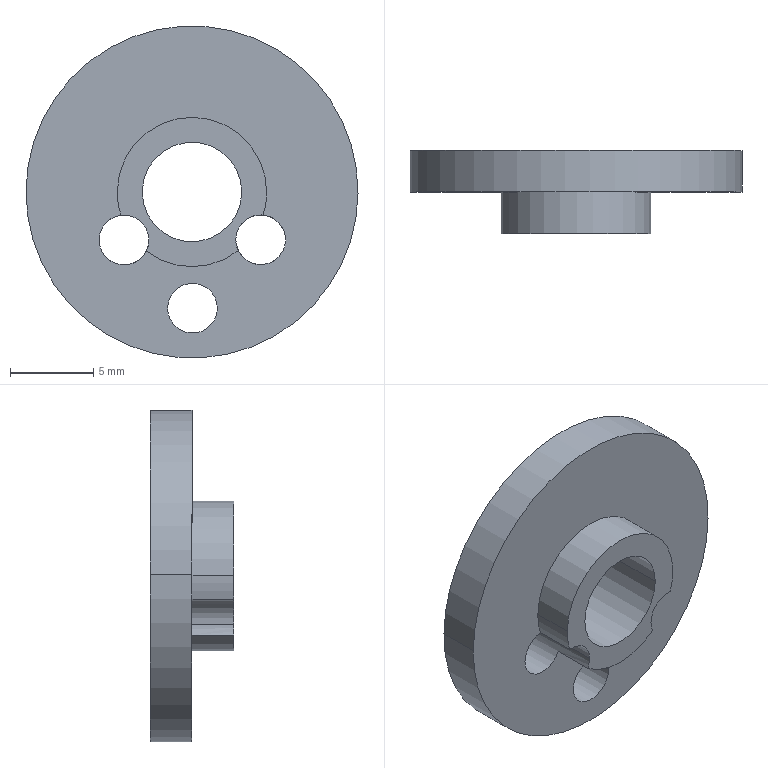Component | SolidWorks | Part6-1 | 1 solid | 17 faces | box 20 x 5 x 20 mm | volume 741 mm3 | cylinder 14 | plane 3 | commonest cylinder face diameters 3 x6 9 x4 20 x2 6 x2 | material 45
build123d program:
from build123d import *

# Parameters (mm, degrees)
SKETCH3_R                = 4.5
SKETCH3_R_2              = 3
BOSS_EXTRUDE1_DEPTH      = 3
BOSS_EXTRUDE2_DEPTH      = 2
BOSS_EXTRUDE2_DEPTH_BACK = 0.5
SKETCH4_R                = 10
SKETCH4_R_2              = 3
SKETCH5_R                = 1.5
CUT_EXTRUDE1_DEPTH       = 16


with BuildPart() as part:
    # Sketch3 → Boss-Extrude1 (new body)
    with BuildSketch(Plane.XY):
        Circle(SKETCH3_R)
        Circle(SKETCH3_R_2, mode=Mode.SUBTRACT)
    extrude(amount=BOSS_EXTRUDE1_DEPTH)

    # Sketch4 → Boss-Extrude2 (add, two sides: drawn at the far end of the back side and taken through both)
    with BuildSketch(Plane.XY.offset(3).offset(-BOSS_EXTRUDE2_DEPTH_BACK)):
        Circle(SKETCH4_R)
        Circle(SKETCH4_R_2, mode=Mode.SUBTRACT)
    extrude(amount=BOSS_EXTRUDE2_DEPTH + BOSS_EXTRUDE2_DEPTH_BACK)

    # Sketch5 → Cut-Extrude1 (cut, through all)
    with BuildSketch(Plane.XY.offset(5)):
        with Locations((4.165, 2.835)):
            Circle(SKETCH5_R)
        with Locations((0.09793, 7)):
            Circle(SKETCH5_R)
        with Locations((0, -1.232)):
            Circle(SKETCH5_R)
        with Locations((-4.067, 2.933)):
            Circle(SKETCH5_R)
    extrude(amount=-CUT_EXTRUDE1_DEPTH, mode=Mode.SUBTRACT)


solid = part.part

# Placed as in the assembly
solid = solid.moved(Location((0, 12.25, 0), (-90, 0, 0.5611)))
STEP:
#1=COLOUR_RGB('',0.7922,0.8196,0.9333);
#2=FILL_AREA_STYLE_COLOUR('',#1);
#3=FILL_AREA_STYLE('',(#2));
#4=SURFACE_STYLE_FILL_AREA(#3);
#5=SURFACE_SIDE_STYLE('',(#4));
#6=SURFACE_STYLE_USAGE(.BOTH.,#5);
#7=PRESENTATION_STYLE_ASSIGNMENT((#6));
#8=CARTESIAN_POINT('',(-0.2203,0.5807,-0.1133));
#9=VERTEX_POINT('',#8);
#10=CARTESIAN_POINT('',(-0.1683,0.5807,-0.05527));
#11=VERTEX_POINT('',#10);
#12=CARTESIAN_POINT('',(-0.1612,0.5807,-0.1139));
#13=DIRECTION('',(-0.,1.,0.));
#14=DIRECTION('',(1.,0.,-0.009793));
#15=AXIS2_PLACEMENT_3D('',#12,#13,#14);
#16=CIRCLE('',#15,0.05906);
#17=EDGE_CURVE('',#9,#11,#16,.T.);
#18=ORIENTED_EDGE('',*,*,#17,.F.);
#19=CARTESIAN_POINT('',(-0.2203,0.6791,-0.1133));
#20=VERTEX_POINT('',#19);
#21=CARTESIAN_POINT('',(-0.2203,0.4823,-0.1133));
#22=DIRECTION('',(-0.,1.,0.));
#23=VECTOR('',#22,39.37);
#24=LINE('',#21,#23);
#25=EDGE_CURVE('',#9,#20,#24,.T.);
#26=ORIENTED_EDGE('',*,*,#25,.T.);
#27=CARTESIAN_POINT('',(-0.1022,0.6791,-0.1145));
#28=VERTEX_POINT('',#27);
#29=CARTESIAN_POINT('',(-0.1612,0.6791,-0.1139));
#30=DIRECTION('',(-0.,1.,0.));
#31=DIRECTION('',(1.,0.,-0.009793));
#32=AXIS2_PLACEMENT_3D('',#29,#30,#31);
#33=CIRCLE('',#32,0.05906);
#34=EDGE_CURVE('',#20,#28,#33,.T.);
#35=ORIENTED_EDGE('',*,*,#34,.T.);
#36=CARTESIAN_POINT('',(-0.1022,0.4823,-0.1145));
#37=VERTEX_POINT('',#36);
#38=CARTESIAN_POINT('',(-0.1022,0.4823,-0.1145));
#39=DIRECTION('',(-0.,1.,0.));
#40=VECTOR('',#39,39.37);
#41=LINE('',#38,#40);
#42=EDGE_CURVE('',#37,#28,#41,.T.);
#43=ORIENTED_EDGE('',*,*,#42,.F.);
#44=CARTESIAN_POINT('',(-0.1683,0.4823,-0.05527));
#45=VERTEX_POINT('',#44);
#46=CARTESIAN_POINT('',(-0.1612,0.4823,-0.1139));
#47=DIRECTION('',(-0.,1.,0.));
#48=DIRECTION('',(1.,0.,-0.009793));
#49=AXIS2_PLACEMENT_3D('',#46,#47,#48);
#50=CIRCLE('',#49,0.05906);
#51=EDGE_CURVE('',#45,#37,#50,.T.);
#52=ORIENTED_EDGE('',*,*,#51,.F.);
#53=CARTESIAN_POINT('',(-0.1683,0.5807,-0.05527));
#54=DIRECTION('',(0.,-1.,-0.));
#55=VECTOR('',#54,39.37);
#56=LINE('',#53,#55);
#57=EDGE_CURVE('',#11,#45,#56,.T.);
#58=ORIENTED_EDGE('',*,*,#57,.F.);
#59=EDGE_LOOP('',(#18,#26,#35,#43,#52,#58));
#60=FACE_OUTER_BOUND('',#59,.T.);
#61=CARTESIAN_POINT('',(-0.1612,0.4823,-0.1139));
#62=DIRECTION('',(-0.,1.,0.));
#63=DIRECTION('',(1.,0.,-0.009793));
#64=AXIS2_PLACEMENT_3D('',#61,#62,#63);
#65=CYLINDRICAL_SURFACE('',#64,0.05906);
#66=ADVANCED_FACE('',(#60),#65,.F.);
#67=CARTESIAN_POINT('',(0.1038,0.4823,-0.1126));
#68=VERTEX_POINT('',#67);
#69=CARTESIAN_POINT('',(0.1686,0.4823,-0.05444));
#70=VERTEX_POINT('',#69);
#71=CARTESIAN_POINT('',(0.1629,0.4823,-0.1132));
#72=DIRECTION('',(-0.,1.,0.));
#73=DIRECTION('',(1.,0.,-0.009793));
#74=AXIS2_PLACEMENT_3D('',#71,#72,#73);
#75=CIRCLE('',#74,0.05906);
#76=EDGE_CURVE('',#68,#70,#75,.T.);
#77=ORIENTED_EDGE('',*,*,#76,.F.);
#78=CARTESIAN_POINT('',(0.1038,0.6791,-0.1126));
#79=VERTEX_POINT('',#78);
#80=CARTESIAN_POINT('',(0.1038,0.4823,-0.1126));
#81=DIRECTION('',(-0.,1.,0.));
#82=VECTOR('',#81,39.37);
#83=LINE('',#80,#82);
#84=EDGE_CURVE('',#68,#79,#83,.T.);
#85=ORIENTED_EDGE('',*,*,#84,.T.);
#86=CARTESIAN_POINT('',(0.2219,0.6791,-0.1138));
#87=VERTEX_POINT('',#86);
#88=CARTESIAN_POINT('',(0.1629,0.6791,-0.1132));
#89=DIRECTION('',(-0.,1.,0.));
#90=DIRECTION('',(1.,0.,-0.009793));
#91=AXIS2_PLACEMENT_3D('',#88,#89,#90);
#92=CIRCLE('',#91,0.05906);
#93=EDGE_CURVE('',#79,#87,#92,.T.);
#94=ORIENTED_EDGE('',*,*,#93,.T.);
#95=CARTESIAN_POINT('',(0.2219,0.5807,-0.1138));
#96=VERTEX_POINT('',#95);
#97=CARTESIAN_POINT('',(0.2219,0.4823,-0.1138));
#98=DIRECTION('',(-0.,1.,0.));
#99=VECTOR('',#98,39.37);
#100=LINE('',#97,#99);
#101=EDGE_CURVE('',#96,#87,#100,.T.);
#102=ORIENTED_EDGE('',*,*,#101,.F.);
#103=CARTESIAN_POINT('',(0.1686,0.5807,-0.05444));
#104=VERTEX_POINT('',#103);
#105=CARTESIAN_POINT('',(0.1629,0.5807,-0.1132));
#106=DIRECTION('',(-0.,1.,0.));
#107=DIRECTION('',(1.,0.,-0.009793));
#108=AXIS2_PLACEMENT_3D('',#105,#106,#107);
#109=CIRCLE('',#108,0.05906);
#110=EDGE_CURVE('',#104,#96,#109,.T.);
#111=ORIENTED_EDGE('',*,*,#110,.F.);
#112=CARTESIAN_POINT('',(0.1686,0.5807,-0.05444));
#113=DIRECTION('',(-0.,1.,0.));
#114=VECTOR('',#113,39.37);
#115=LINE('',#112,#114);
#116=EDGE_CURVE('',#70,#104,#115,.T.);
#117=ORIENTED_EDGE('',*,*,#116,.F.);
#118=EDGE_LOOP('',(#77,#85,#94,#102,#111,#117));
#119=FACE_OUTER_BOUND('',#118,.T.);
#120=CARTESIAN_POINT('',(0.1629,0.4823,-0.1132));
#121=DIRECTION('',(-0.,1.,0.));
#122=DIRECTION('',(1.,0.,-0.009793));
#123=AXIS2_PLACEMENT_3D('',#120,#121,#122);
#124=CYLINDRICAL_SURFACE('',#123,0.05906);
#125=ADVANCED_FACE('',(#119),#124,.F.);
#126=CARTESIAN_POINT('',(-0.0579,0.5807,-0.275));
#127=VERTEX_POINT('',#126);
#128=CARTESIAN_POINT('',(0.06021,0.5807,-0.2762));
#129=VERTEX_POINT('',#128);
#130=CARTESIAN_POINT('',(0.001157,0.5807,-0.2756));
#131=DIRECTION('',(-0.,1.,0.));
#132=DIRECTION('',(1.,0.,-0.009793));
#133=AXIS2_PLACEMENT_3D('',#130,#131,#132);
#134=CIRCLE('',#133,0.05906);
#135=EDGE_CURVE('',#127,#129,#134,.T.);
#136=ORIENTED_EDGE('',*,*,#135,.F.);
#137=CARTESIAN_POINT('',(-0.0579,0.6791,-0.275));
#138=VERTEX_POINT('',#137);
#139=CARTESIAN_POINT('',(-0.0579,0.4823,-0.275));
#140=DIRECTION('',(-0.,1.,0.));
#141=VECTOR('',#140,39.37);
#142=LINE('',#139,#141);
#143=EDGE_CURVE('',#127,#138,#142,.T.);
#144=ORIENTED_EDGE('',*,*,#143,.T.);
#145=CARTESIAN_POINT('',(0.06021,0.6791,-0.2762));
#146=VERTEX_POINT('',#145);
#147=CARTESIAN_POINT('',(0.001157,0.6791,-0.2756));
#148=DIRECTION('',(-0.,1.,0.));
#149=DIRECTION('',(1.,0.,-0.009793));
#150=AXIS2_PLACEMENT_3D('',#147,#148,#149);
#151=CIRCLE('',#150,0.05906);
#152=EDGE_CURVE('',#138,#146,#151,.T.);
#153=ORIENTED_EDGE('',*,*,#152,.T.);
#154=CARTESIAN_POINT('',(0.06021,0.4823,-0.2762));
#155=DIRECTION('',(-0.,1.,0.));
#156=VECTOR('',#155,39.37);
#157=LINE('',#154,#156);
#158=EDGE_CURVE('',#129,#146,#157,.T.);
#159=ORIENTED_EDGE('',*,*,#158,.F.);
#160=EDGE_LOOP('',(#136,#144,#153,#159));
#161=FACE_OUTER_BOUND('',#160,.T.);
#162=CARTESIAN_POINT('',(0.001157,0.4823,-0.2756));
#163=DIRECTION('',(-0.,1.,0.));
#164=DIRECTION('',(1.,0.,-0.009793));
#165=AXIS2_PLACEMENT_3D('',#162,#163,#164);
#166=CYLINDRICAL_SURFACE('',#165,0.05906);
#167=ADVANCED_FACE('',(#161),#166,.F.);
#168=CARTESIAN_POINT('',(0.3937,0.5807,-0.003856));
#169=VERTEX_POINT('',#168);
#170=CARTESIAN_POINT('',(-0.3937,0.5807,0.003856));
#171=VERTEX_POINT('',#170);
#172=CARTESIAN_POINT('',(-0.,0.5807,-0.));
#173=DIRECTION('',(-0.,1.,0.));
#174=DIRECTION('',(1.,0.,-0.009793));
#175=AXIS2_PLACEMENT_3D('',#172,#173,#174);
#176=CIRCLE('',#175,0.3937);
#177=EDGE_CURVE('',#169,#171,#176,.T.);
#178=ORIENTED_EDGE('',*,*,#177,.T.);
#179=CARTESIAN_POINT('',(-0.3937,0.6791,0.003856));
#180=VERTEX_POINT('',#179);
#181=CARTESIAN_POINT('',(-0.3937,0.5807,0.003856));
#182=DIRECTION('',(-0.,1.,0.));
#183=VECTOR('',#182,39.37);
#184=LINE('',#181,#183);
#185=EDGE_CURVE('',#171,#180,#184,.T.);
#186=ORIENTED_EDGE('',*,*,#185,.T.);
#187=CARTESIAN_POINT('',(0.3937,0.6791,-0.003856));
#188=VERTEX_POINT('',#187);
#189=CARTESIAN_POINT('',(-0.,0.6791,-0.));
#190=DIRECTION('',(-0.,1.,0.));
#191=DIRECTION('',(1.,0.,-0.009793));
#192=AXIS2_PLACEMENT_3D('',#189,#190,#191);
#193=CIRCLE('',#192,0.3937);
#194=EDGE_CURVE('',#188,#180,#193,.T.);
#195=ORIENTED_EDGE('',*,*,#194,.F.);
#196=CARTESIAN_POINT('',(0.3937,0.5807,-0.003856));
#197=DIRECTION('',(-0.,1.,0.));
#198=VECTOR('',#197,39.37);
#199=LINE('',#196,#198);
#200=EDGE_CURVE('',#169,#188,#199,.T.);
#201=ORIENTED_EDGE('',*,*,#200,.F.);
#202=EDGE_LOOP('',(#178,#186,#195,#201));
#203=FACE_OUTER_BOUND('',#202,.T.);
#204=CARTESIAN_POINT('',(-0.,0.5807,-0.));
#205=DIRECTION('',(-0.,1.,0.));
#206=DIRECTION('',(1.,0.,-0.009793));
#207=AXIS2_PLACEMENT_3D('',#204,#205,#206);
#208=CYLINDRICAL_SURFACE('',#207,0.3937);
#209=ADVANCED_FACE('',(#203),#208,.T.);
#210=CARTESIAN_POINT('',(-0.1181,0.6791,0.001157));
#211=VERTEX_POINT('',#210);
#212=CARTESIAN_POINT('',(0.1181,0.6791,-0.001157));
#213=VERTEX_POINT('',#212);
#214=CARTESIAN_POINT('',(-0.,0.6791,-0.));
#215=DIRECTION('',(-0.,1.,0.));
#216=DIRECTION('',(1.,0.,-0.009793));
#217=AXIS2_PLACEMENT_3D('',#214,#215,#216);
#218=CIRCLE('',#217,0.1181);
#219=EDGE_CURVE('',#211,#213,#218,.T.);
#220=ORIENTED_EDGE('',*,*,#219,.T.);
#221=CARTESIAN_POINT('',(0.1181,0.4823,-0.001157));
#222=VERTEX_POINT('',#221);
#223=CARTESIAN_POINT('',(0.1181,0.6004,-0.001157));
#224=DIRECTION('',(0.,-1.,-0.));
#225=VECTOR('',#224,39.37);
#226=LINE('',#223,#225);
#227=EDGE_CURVE('',#213,#222,#226,.T.);
#228=ORIENTED_EDGE('',*,*,#227,.T.);
#229=CARTESIAN_POINT('',(-0.1181,0.4823,0.001157));
#230=VERTEX_POINT('',#229);
#231=CARTESIAN_POINT('',(-0.,0.4823,-0.));
#232=DIRECTION('',(-0.,1.,0.));
#233=DIRECTION('',(1.,0.,-0.009793));
#234=AXIS2_PLACEMENT_3D('',#231,#232,#233);
#235=CIRCLE('',#234,0.1181);
#236=EDGE_CURVE('',#230,#222,#235,.T.);
#237=ORIENTED_EDGE('',*,*,#236,.F.);
#238=CARTESIAN_POINT('',(-0.1181,0.6004,0.001157));
#239=DIRECTION('',(0.,-1.,-0.));
#240=VECTOR('',#239,39.37);
#241=LINE('',#238,#240);
#242=EDGE_CURVE('',#211,#230,#241,.T.);
#243=ORIENTED_EDGE('',*,*,#242,.F.);
#244=EDGE_LOOP('',(#220,#228,#237,#243));
#245=FACE_OUTER_BOUND('',#244,.T.);
#246=CARTESIAN_POINT('',(-0.,0.6004,-0.));
#247=DIRECTION('',(0.,-1.,-0.));
#248=DIRECTION('',(-1.,0.,0.009793));
#249=AXIS2_PLACEMENT_3D('',#246,#247,#248);
#250=CYLINDRICAL_SURFACE('',#249,0.1181);
#251=ADVANCED_FACE('',(#245),#250,.F.);
#252=CARTESIAN_POINT('',(0.1772,0.5807,-0.001735));
#253=VERTEX_POINT('',#252);
#254=CARTESIAN_POINT('',(-0.,0.5807,-0.));
#255=DIRECTION('',(-0.,1.,0.));
#256=DIRECTION('',(1.,0.,-0.009793));
#257=AXIS2_PLACEMENT_3D('',#254,#255,#256);
#258=CIRCLE('',#257,0.1772);
#259=EDGE_CURVE('',#253,#104,#258,.T.);
#260=ORIENTED_EDGE('',*,*,#259,.F.);
#261=CARTESIAN_POINT('',(0.1772,0.4823,-0.001735));
#262=VERTEX_POINT('',#261);
#263=CARTESIAN_POINT('',(0.1772,0.6004,-0.001735));
#264=DIRECTION('',(0.,-1.,-0.));
#265=VECTOR('',#264,39.37);
#266=LINE('',#263,#265);
#267=EDGE_CURVE('',#253,#262,#266,.T.);
#268=ORIENTED_EDGE('',*,*,#267,.T.);
#269=CARTESIAN_POINT('',(-0.,0.4823,-0.));
#270=DIRECTION('',(-0.,1.,0.));
#271=DIRECTION('',(1.,0.,-0.009793));
#272=AXIS2_PLACEMENT_3D('',#269,#270,#271);
#273=CIRCLE('',#272,0.1772);
#274=EDGE_CURVE('',#262,#70,#273,.T.);
#275=ORIENTED_EDGE('',*,*,#274,.T.);
#276=ORIENTED_EDGE('',*,*,#116,.T.);
#277=EDGE_LOOP('',(#260,#268,#275,#276));
#278=FACE_OUTER_BOUND('',#277,.T.);
#279=CARTESIAN_POINT('',(-0.,0.6004,-0.));
#280=DIRECTION('',(0.,-1.,-0.));
#281=DIRECTION('',(-1.,0.,0.009793));
#282=AXIS2_PLACEMENT_3D('',#279,#280,#281);
#283=CYLINDRICAL_SURFACE('',#282,0.1772);
#284=ADVANCED_FACE('',(#278),#283,.T.);
#285=ORIENTED_EDGE('',*,*,#267,.F.);
#286=CARTESIAN_POINT('',(-0.1772,0.5807,0.001735));
#287=VERTEX_POINT('',#286);
#288=CARTESIAN_POINT('',(-0.,0.5807,-0.));
#289=DIRECTION('',(-0.,1.,0.));
#290=DIRECTION('',(1.,0.,-0.009793));
#291=AXIS2_PLACEMENT_3D('',#288,#289,#290);
#292=CIRCLE('',#291,0.1772);
#293=EDGE_CURVE('',#287,#253,#292,.T.);
#294=ORIENTED_EDGE('',*,*,#293,.F.);
#295=CARTESIAN_POINT('',(-0.1772,0.4823,0.001735));
#296=VERTEX_POINT('',#295);
#297=CARTESIAN_POINT('',(-0.1772,0.6004,0.001735));
#298=DIRECTION('',(0.,-1.,-0.));
#299=VECTOR('',#298,39.37);
#300=LINE('',#297,#299);
#301=EDGE_CURVE('',#287,#296,#300,.T.);
#302=ORIENTED_EDGE('',*,*,#301,.T.);
#303=CARTESIAN_POINT('',(-0.,0.4823,-0.));
#304=DIRECTION('',(-0.,1.,0.));
#305=DIRECTION('',(1.,0.,-0.009793));
#306=AXIS2_PLACEMENT_3D('',#303,#304,#305);
#307=CIRCLE('',#306,0.1772);
#308=EDGE_CURVE('',#296,#262,#307,.T.);
#309=ORIENTED_EDGE('',*,*,#308,.T.);
#310=EDGE_LOOP('',(#285,#294,#302,#309));
#311=FACE_OUTER_BOUND('',#310,.T.);
#312=CARTESIAN_POINT('',(-0.,0.6004,-0.));
#313=DIRECTION('',(0.,-1.,-0.));
#314=DIRECTION('',(-1.,0.,0.009793));
#315=AXIS2_PLACEMENT_3D('',#312,#313,#314);
#316=CYLINDRICAL_SURFACE('',#315,0.1772);
#317=ADVANCED_FACE('',(#311),#316,.T.);
#318=CARTESIAN_POINT('',(0.1098,0.4823,-0.1391));
#319=VERTEX_POINT('',#318);
#320=CARTESIAN_POINT('',(-0.1084,0.4823,-0.1402));
#321=VERTEX_POINT('',#320);
#322=CARTESIAN_POINT('',(-0.,0.4823,-0.));
#323=DIRECTION('',(-0.,1.,0.));
#324=DIRECTION('',(1.,0.,-0.009793));
#325=AXIS2_PLACEMENT_3D('',#322,#323,#324);
#326=CIRCLE('',#325,0.1772);
#327=EDGE_CURVE('',#319,#321,#326,.T.);
#328=ORIENTED_EDGE('',*,*,#327,.T.);
#329=CARTESIAN_POINT('',(-0.1084,0.5807,-0.1402));
#330=VERTEX_POINT('',#329);
#331=CARTESIAN_POINT('',(-0.1084,0.5807,-0.1402));
#332=DIRECTION('',(-0.,1.,0.));
#333=VECTOR('',#332,39.37);
#334=LINE('',#331,#333);
#335=EDGE_CURVE('',#321,#330,#334,.T.);
#336=ORIENTED_EDGE('',*,*,#335,.T.);
#337=CARTESIAN_POINT('',(0.1098,0.5807,-0.1391));
#338=VERTEX_POINT('',#337);
#339=CARTESIAN_POINT('',(-0.,0.5807,-0.));
#340=DIRECTION('',(-0.,1.,0.));
#341=DIRECTION('',(1.,0.,-0.009793));
#342=AXIS2_PLACEMENT_3D('',#339,#340,#341);
#343=CIRCLE('',#342,0.1772);
#344=EDGE_CURVE('',#338,#330,#343,.T.);
#345=ORIENTED_EDGE('',*,*,#344,.F.);
#346=CARTESIAN_POINT('',(0.1098,0.5807,-0.1391));
#347=DIRECTION('',(0.,-1.,-0.));
#348=VECTOR('',#347,39.37);
#349=LINE('',#346,#348);
#350=EDGE_CURVE('',#338,#319,#349,.T.);
#351=ORIENTED_EDGE('',*,*,#350,.T.);
#352=EDGE_LOOP('',(#328,#336,#345,#351));
#353=FACE_OUTER_BOUND('',#352,.T.);
#354=CARTESIAN_POINT('',(-0.,0.6004,-0.));
#355=DIRECTION('',(0.,-1.,-0.));
#356=DIRECTION('',(-1.,0.,0.009793));
#357=AXIS2_PLACEMENT_3D('',#354,#355,#356);
#358=CYLINDRICAL_SURFACE('',#357,0.1772);
#359=ADVANCED_FACE('',(#353),#358,.T.);
#360=ORIENTED_EDGE('',*,*,#301,.F.);
#361=CARTESIAN_POINT('',(-0.,0.5807,-0.));
#362=DIRECTION('',(-0.,1.,0.));
#363=DIRECTION('',(1.,0.,-0.009793));
#364=AXIS2_PLACEMENT_3D('',#361,#362,#363);
#365=CIRCLE('',#364,0.1772);
#366=EDGE_CURVE('',#11,#287,#365,.T.);
#367=ORIENTED_EDGE('',*,*,#366,.F.);
#368=ORIENTED_EDGE('',*,*,#57,.T.);
#369=CARTESIAN_POINT('',(-0.,0.4823,-0.));
#370=DIRECTION('',(-0.,1.,0.));
#371=DIRECTION('',(1.,0.,-0.009793));
#372=AXIS2_PLACEMENT_3D('',#369,#370,#371);
#373=CIRCLE('',#372,0.1772);
#374=EDGE_CURVE('',#45,#296,#373,.T.);
#375=ORIENTED_EDGE('',*,*,#374,.T.);
#376=EDGE_LOOP('',(#360,#367,#368,#375));
#377=FACE_OUTER_BOUND('',#376,.T.);
#378=CARTESIAN_POINT('',(-0.,0.6004,-0.));
#379=DIRECTION('',(0.,-1.,-0.));
#380=DIRECTION('',(-1.,0.,0.009793));
#381=AXIS2_PLACEMENT_3D('',#378,#379,#380);
#382=CYLINDRICAL_SURFACE('',#381,0.1772);
#383=ADVANCED_FACE('',(#377),#382,.T.);
#384=ORIENTED_EDGE('',*,*,#374,.F.);
#385=ORIENTED_EDGE('',*,*,#51,.T.);
#386=CARTESIAN_POINT('',(-0.1612,0.4823,-0.1139));
#387=DIRECTION('',(-0.,1.,0.));
#388=DIRECTION('',(1.,0.,-0.009793));
#389=AXIS2_PLACEMENT_3D('',#386,#387,#388);
#390=CIRCLE('',#389,0.05906);
#391=EDGE_CURVE('',#37,#321,#390,.T.);
#392=ORIENTED_EDGE('',*,*,#391,.T.);
#393=ORIENTED_EDGE('',*,*,#327,.F.);
#394=CARTESIAN_POINT('',(0.1629,0.4823,-0.1132));
#395=DIRECTION('',(-0.,1.,0.));
#396=DIRECTION('',(1.,0.,-0.009793));
#397=AXIS2_PLACEMENT_3D('',#394,#395,#396);
#398=CIRCLE('',#397,0.05906);
#399=EDGE_CURVE('',#319,#68,#398,.T.);
#400=ORIENTED_EDGE('',*,*,#399,.T.);
#401=ORIENTED_EDGE('',*,*,#76,.T.);
#402=ORIENTED_EDGE('',*,*,#274,.F.);
#403=ORIENTED_EDGE('',*,*,#308,.F.);
#404=EDGE_LOOP('',(#384,#385,#392,#393,#400,#401,#402,#403));
#405=FACE_OUTER_BOUND('',#404,.T.);
#406=ORIENTED_EDGE('',*,*,#236,.T.);
#407=CARTESIAN_POINT('',(-0.,0.4823,-0.));
#408=DIRECTION('',(-0.,1.,0.));
#409=DIRECTION('',(1.,0.,-0.009793));
#410=AXIS2_PLACEMENT_3D('',#407,#408,#409);
#411=CIRCLE('',#410,0.1181);
#412=EDGE_CURVE('',#222,#230,#411,.T.);
#413=ORIENTED_EDGE('',*,*,#412,.T.);
#414=EDGE_LOOP('',(#406,#413));
#415=FACE_BOUND('',#414,.T.);
#416=CARTESIAN_POINT('',(-0.,0.4823,-0.));
#417=DIRECTION('',(-0.,1.,0.));
#418=DIRECTION('',(1.,0.,-0.009793));
#419=AXIS2_PLACEMENT_3D('',#416,#417,#418);
#420=PLANE('',#419);
#421=ADVANCED_FACE('',(#405,#415),#420,.F.);
#422=ORIENTED_EDGE('',*,*,#227,.F.);
#423=CARTESIAN_POINT('',(-0.,0.6791,-0.));
#424=DIRECTION('',(-0.,1.,0.));
#425=DIRECTION('',(1.,0.,-0.009793));
#426=AXIS2_PLACEMENT_3D('',#423,#424,#425);
#427=CIRCLE('',#426,0.1181);
#428=EDGE_CURVE('',#213,#211,#427,.T.);
#429=ORIENTED_EDGE('',*,*,#428,.T.);
#430=ORIENTED_EDGE('',*,*,#242,.T.);
#431=ORIENTED_EDGE('',*,*,#412,.F.);
#432=EDGE_LOOP('',(#422,#429,#430,#431));
#433=FACE_OUTER_BOUND('',#432,.T.);
#434=CARTESIAN_POINT('',(-0.,0.6004,-0.));
#435=DIRECTION('',(0.,-1.,-0.));
#436=DIRECTION('',(-1.,0.,0.009793));
#437=AXIS2_PLACEMENT_3D('',#434,#435,#436);
#438=CYLINDRICAL_SURFACE('',#437,0.1181);
#439=ADVANCED_FACE('',(#433),#438,.F.);
#440=CARTESIAN_POINT('',(0.001157,0.5807,-0.2756));
#441=DIRECTION('',(-0.,1.,0.));
#442=DIRECTION('',(1.,0.,-0.009793));
#443=AXIS2_PLACEMENT_3D('',#440,#441,#442);
#444=CIRCLE('',#443,0.05906);
#445=EDGE_CURVE('',#129,#127,#444,.T.);
#446=ORIENTED_EDGE('',*,*,#445,.T.);
#447=ORIENTED_EDGE('',*,*,#135,.T.);
#448=EDGE_LOOP('',(#446,#447));
#449=FACE_BOUND('',#448,.T.);
#450=ORIENTED_EDGE('',*,*,#177,.F.);
#451=CARTESIAN_POINT('',(-0.,0.5807,-0.));
#452=DIRECTION('',(-0.,1.,0.));
#453=DIRECTION('',(1.,0.,-0.009793));
#454=AXIS2_PLACEMENT_3D('',#451,#452,#453);
#455=CIRCLE('',#454,0.3937);
#456=EDGE_CURVE('',#171,#169,#455,.T.);
#457=ORIENTED_EDGE('',*,*,#456,.F.);
#458=EDGE_LOOP('',(#450,#457));
#459=FACE_OUTER_BOUND('',#458,.T.);
#460=ORIENTED_EDGE('',*,*,#344,.T.);
#461=CARTESIAN_POINT('',(-0.1612,0.5807,-0.1139));
#462=DIRECTION('',(-0.,1.,0.));
#463=DIRECTION('',(1.,0.,-0.009793));
#464=AXIS2_PLACEMENT_3D('',#461,#462,#463);
#465=CIRCLE('',#464,0.05906);
#466=EDGE_CURVE('',#330,#9,#465,.T.);
#467=ORIENTED_EDGE('',*,*,#466,.T.);
#468=ORIENTED_EDGE('',*,*,#17,.T.);
#469=ORIENTED_EDGE('',*,*,#366,.T.);
#470=ORIENTED_EDGE('',*,*,#293,.T.);
#471=ORIENTED_EDGE('',*,*,#259,.T.);
#472=ORIENTED_EDGE('',*,*,#110,.T.);
#473=CARTESIAN_POINT('',(0.1629,0.5807,-0.1132));
#474=DIRECTION('',(-0.,1.,0.));
#475=DIRECTION('',(1.,0.,-0.009793));
#476=AXIS2_PLACEMENT_3D('',#473,#474,#475);
#477=CIRCLE('',#476,0.05906);
#478=EDGE_CURVE('',#96,#338,#477,.T.);
#479=ORIENTED_EDGE('',*,*,#478,.T.);
#480=EDGE_LOOP('',(#460,#467,#468,#469,#470,#471,#472,#479));
#481=FACE_BOUND('',#480,.T.);
#482=CARTESIAN_POINT('',(-0.,0.5807,-0.));
#483=DIRECTION('',(-0.,1.,0.));
#484=DIRECTION('',(1.,0.,-0.009793));
#485=AXIS2_PLACEMENT_3D('',#482,#483,#484);
#486=PLANE('',#485);
#487=ADVANCED_FACE('',(#449,#459,#481),#486,.F.);
#488=ORIENTED_EDGE('',*,*,#185,.F.);
#489=ORIENTED_EDGE('',*,*,#456,.T.);
#490=ORIENTED_EDGE('',*,*,#200,.T.);
#491=CARTESIAN_POINT('',(-0.,0.6791,-0.));
#492=DIRECTION('',(-0.,1.,0.));
#493=DIRECTION('',(1.,0.,-0.009793));
#494=AXIS2_PLACEMENT_3D('',#491,#492,#493);
#495=CIRCLE('',#494,0.3937);
#496=EDGE_CURVE('',#180,#188,#495,.T.);
#497=ORIENTED_EDGE('',*,*,#496,.F.);
#498=EDGE_LOOP('',(#488,#489,#490,#497));
#499=FACE_OUTER_BOUND('',#498,.T.);
#500=CARTESIAN_POINT('',(-0.,0.5807,-0.));
#501=DIRECTION('',(-0.,1.,0.));
#502=DIRECTION('',(1.,0.,-0.009793));
#503=AXIS2_PLACEMENT_3D('',#500,#501,#502);
#504=CYLINDRICAL_SURFACE('',#503,0.3937);
#505=ADVANCED_FACE('',(#499),#504,.T.);
#506=CARTESIAN_POINT('',(-0.1612,0.6791,-0.1139));
#507=DIRECTION('',(-0.,1.,0.));
#508=DIRECTION('',(1.,0.,-0.009793));
#509=AXIS2_PLACEMENT_3D('',#506,#507,#508);
#510=CIRCLE('',#509,0.05906);
#511=EDGE_CURVE('',#28,#20,#510,.T.);
#512=ORIENTED_EDGE('',*,*,#511,.F.);
#513=ORIENTED_EDGE('',*,*,#34,.F.);
#514=EDGE_LOOP('',(#512,#513));
#515=FACE_BOUND('',#514,.T.);
#516=CARTESIAN_POINT('',(0.1629,0.6791,-0.1132));
#517=DIRECTION('',(-0.,1.,0.));
#518=DIRECTION('',(1.,0.,-0.009793));
#519=AXIS2_PLACEMENT_3D('',#516,#517,#518);
#520=CIRCLE('',#519,0.05906);
#521=EDGE_CURVE('',#87,#79,#520,.T.);
#522=ORIENTED_EDGE('',*,*,#521,.F.);
#523=ORIENTED_EDGE('',*,*,#93,.F.);
#524=EDGE_LOOP('',(#522,#523));
#525=FACE_BOUND('',#524,.T.);
#526=CARTESIAN_POINT('',(0.001157,0.6791,-0.2756));
#527=DIRECTION('',(-0.,1.,0.));
#528=DIRECTION('',(1.,0.,-0.009793));
#529=AXIS2_PLACEMENT_3D('',#526,#527,#528);
#530=CIRCLE('',#529,0.05906);
#531=EDGE_CURVE('',#146,#138,#530,.T.);
#532=ORIENTED_EDGE('',*,*,#531,.F.);
#533=ORIENTED_EDGE('',*,*,#152,.F.);
#534=EDGE_LOOP('',(#532,#533));
#535=FACE_BOUND('',#534,.T.);
#536=ORIENTED_EDGE('',*,*,#194,.T.);
#537=ORIENTED_EDGE('',*,*,#496,.T.);
#538=EDGE_LOOP('',(#536,#537));
#539=FACE_OUTER_BOUND('',#538,.T.);
#540=ORIENTED_EDGE('',*,*,#219,.F.);
#541=ORIENTED_EDGE('',*,*,#428,.F.);
#542=EDGE_LOOP('',(#540,#541));
#543=FACE_BOUND('',#542,.T.);
#544=CARTESIAN_POINT('',(-0.,0.6791,-0.));
#545=DIRECTION('',(-0.,1.,0.));
#546=DIRECTION('',(1.,0.,-0.009793));
#547=AXIS2_PLACEMENT_3D('',#544,#545,#546);
#548=PLANE('',#547);
#549=ADVANCED_FACE('',(#515,#525,#535,#539,#543),#548,.T.);
#550=ORIENTED_EDGE('',*,*,#143,.F.);
#551=ORIENTED_EDGE('',*,*,#445,.F.);
#552=ORIENTED_EDGE('',*,*,#158,.T.);
#553=ORIENTED_EDGE('',*,*,#531,.T.);
#554=EDGE_LOOP('',(#550,#551,#552,#553));
#555=FACE_OUTER_BOUND('',#554,.T.);
#556=CARTESIAN_POINT('',(0.001157,0.4823,-0.2756));
#557=DIRECTION('',(-0.,1.,0.));
#558=DIRECTION('',(1.,0.,-0.009793));
#559=AXIS2_PLACEMENT_3D('',#556,#557,#558);
#560=CYLINDRICAL_SURFACE('',#559,0.05906);
#561=ADVANCED_FACE('',(#555),#560,.F.);
#562=ORIENTED_EDGE('',*,*,#84,.F.);
#563=ORIENTED_EDGE('',*,*,#399,.F.);
#564=ORIENTED_EDGE('',*,*,#350,.F.);
#565=ORIENTED_EDGE('',*,*,#478,.F.);
#566=ORIENTED_EDGE('',*,*,#101,.T.);
#567=ORIENTED_EDGE('',*,*,#521,.T.);
#568=EDGE_LOOP('',(#562,#563,#564,#565,#566,#567));
#569=FACE_OUTER_BOUND('',#568,.T.);
#570=CARTESIAN_POINT('',(0.1629,0.4823,-0.1132));
#571=DIRECTION('',(-0.,1.,0.));
#572=DIRECTION('',(1.,0.,-0.009793));
#573=AXIS2_PLACEMENT_3D('',#570,#571,#572);
#574=CYLINDRICAL_SURFACE('',#573,0.05906);
#575=ADVANCED_FACE('',(#569),#574,.F.);
#576=ORIENTED_EDGE('',*,*,#25,.F.);
#577=ORIENTED_EDGE('',*,*,#466,.F.);
#578=ORIENTED_EDGE('',*,*,#335,.F.);
#579=ORIENTED_EDGE('',*,*,#391,.F.);
#580=ORIENTED_EDGE('',*,*,#42,.T.);
#581=ORIENTED_EDGE('',*,*,#511,.T.);
#582=EDGE_LOOP('',(#576,#577,#578,#579,#580,#581));
#583=FACE_OUTER_BOUND('',#582,.T.);
#584=CARTESIAN_POINT('',(-0.1612,0.4823,-0.1139));
#585=DIRECTION('',(-0.,1.,0.));
#586=DIRECTION('',(1.,0.,-0.009793));
#587=AXIS2_PLACEMENT_3D('',#584,#585,#586);
#588=CYLINDRICAL_SURFACE('',#587,0.05906);
#589=ADVANCED_FACE('',(#583),#588,.F.);
#590=CLOSED_SHELL('',(#66,#125,#167,#209,#251,#284,#317,#359,#383,#421,#439,#487,#505,#549,#561,#575,#589));
#591=MANIFOLD_SOLID_BREP('',#590);
#592=STYLED_ITEM('',(#7),#591);
#593=PRESENTATION_LAYER_ASSIGNMENT('','',(#592));
#594=(LENGTH_UNIT()NAMED_UNIT(*)SI_UNIT($,.METRE.));
#595=LENGTH_MEASURE_WITH_UNIT(LENGTH_MEASURE(0.0254),#594);
#596=DIMENSIONAL_EXPONENTS(1.,0.,0.,0.,0.,0.,0.);
#597=(CONVERSION_BASED_UNIT('',#595)LENGTH_UNIT()NAMED_UNIT(#596));
#598=UNCERTAINTY_MEASURE_WITH_UNIT(LENGTH_MEASURE(0.00001),#597,'','');
#599=(NAMED_UNIT(*)PLANE_ANGLE_UNIT()SI_UNIT($,.RADIAN.));
#600=(NAMED_UNIT(*)SI_UNIT($,.STERADIAN.)SOLID_ANGLE_UNIT());
#601=(GEOMETRIC_REPRESENTATION_CONTEXT(3)GLOBAL_UNCERTAINTY_ASSIGNED_CONTEXT((#598))GLOBAL_UNIT_ASSIGNED_CONTEXT((#597,#599,#600))REPRESENTATION_CONTEXT('',''));
#602=MECHANICAL_DESIGN_GEOMETRIC_PRESENTATION_REPRESENTATION('',(#592),#601);
#603=CARTESIAN_POINT('',(0.,0.,0.));
#604=DIRECTION('',(0.,0.,1.));
#605=DIRECTION('',(1.,0.,0.));
#606=AXIS2_PLACEMENT_3D('',#603,#604,#605);
#607=(LENGTH_UNIT()NAMED_UNIT(*)SI_UNIT($,.METRE.));
#608=LENGTH_MEASURE_WITH_UNIT(LENGTH_MEASURE(0.0254),#607);
#609=DIMENSIONAL_EXPONENTS(1.,0.,0.,0.,0.,0.,0.);
#610=(CONVERSION_BASED_UNIT('',#608)LENGTH_UNIT()NAMED_UNIT(#609));
#611=UNCERTAINTY_MEASURE_WITH_UNIT(LENGTH_MEASURE(0.00001),#610,'','');
#612=(NAMED_UNIT(*)PLANE_ANGLE_UNIT()SI_UNIT($,.RADIAN.));
#613=(NAMED_UNIT(*)SI_UNIT($,.STERADIAN.)SOLID_ANGLE_UNIT());
#614=(GEOMETRIC_REPRESENTATION_CONTEXT(3)GLOBAL_UNCERTAINTY_ASSIGNED_CONTEXT((#611))GLOBAL_UNIT_ASSIGNED_CONTEXT((#610,#612,#613))REPRESENTATION_CONTEXT('',''));
#615=ADVANCED_BREP_SHAPE_REPRESENTATION('',(#591,#606),#614);